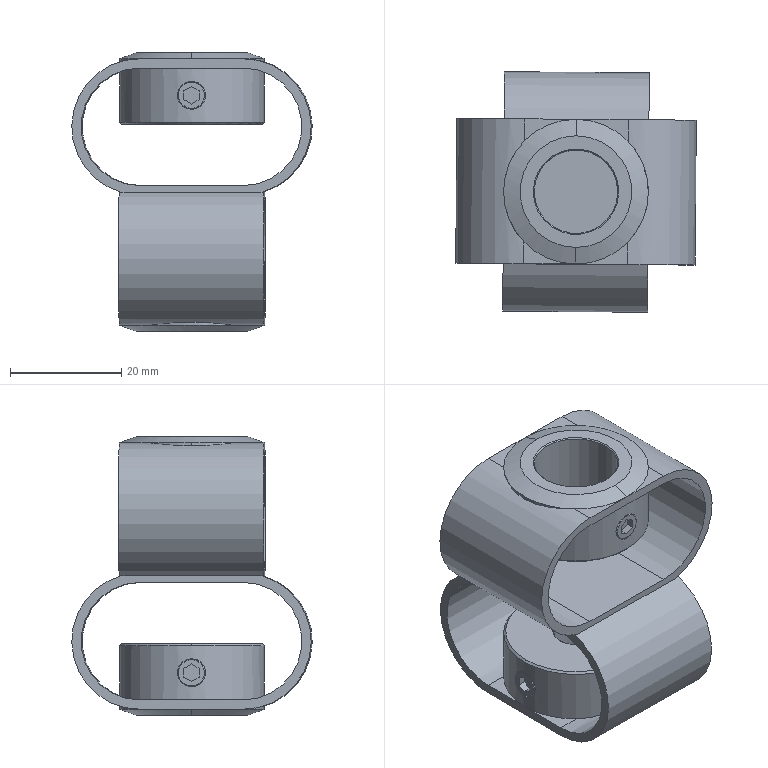Component | SolidWorks | 12ACoupling-1 | 1 solid | 124 faces | volume 17510 mm3 | plane 58 | cylinder 42 | cone 24 | commonest cylinder face diameters 5 x20 26 x10 24.42 x4 21.087 x4 15 x2 8 x2